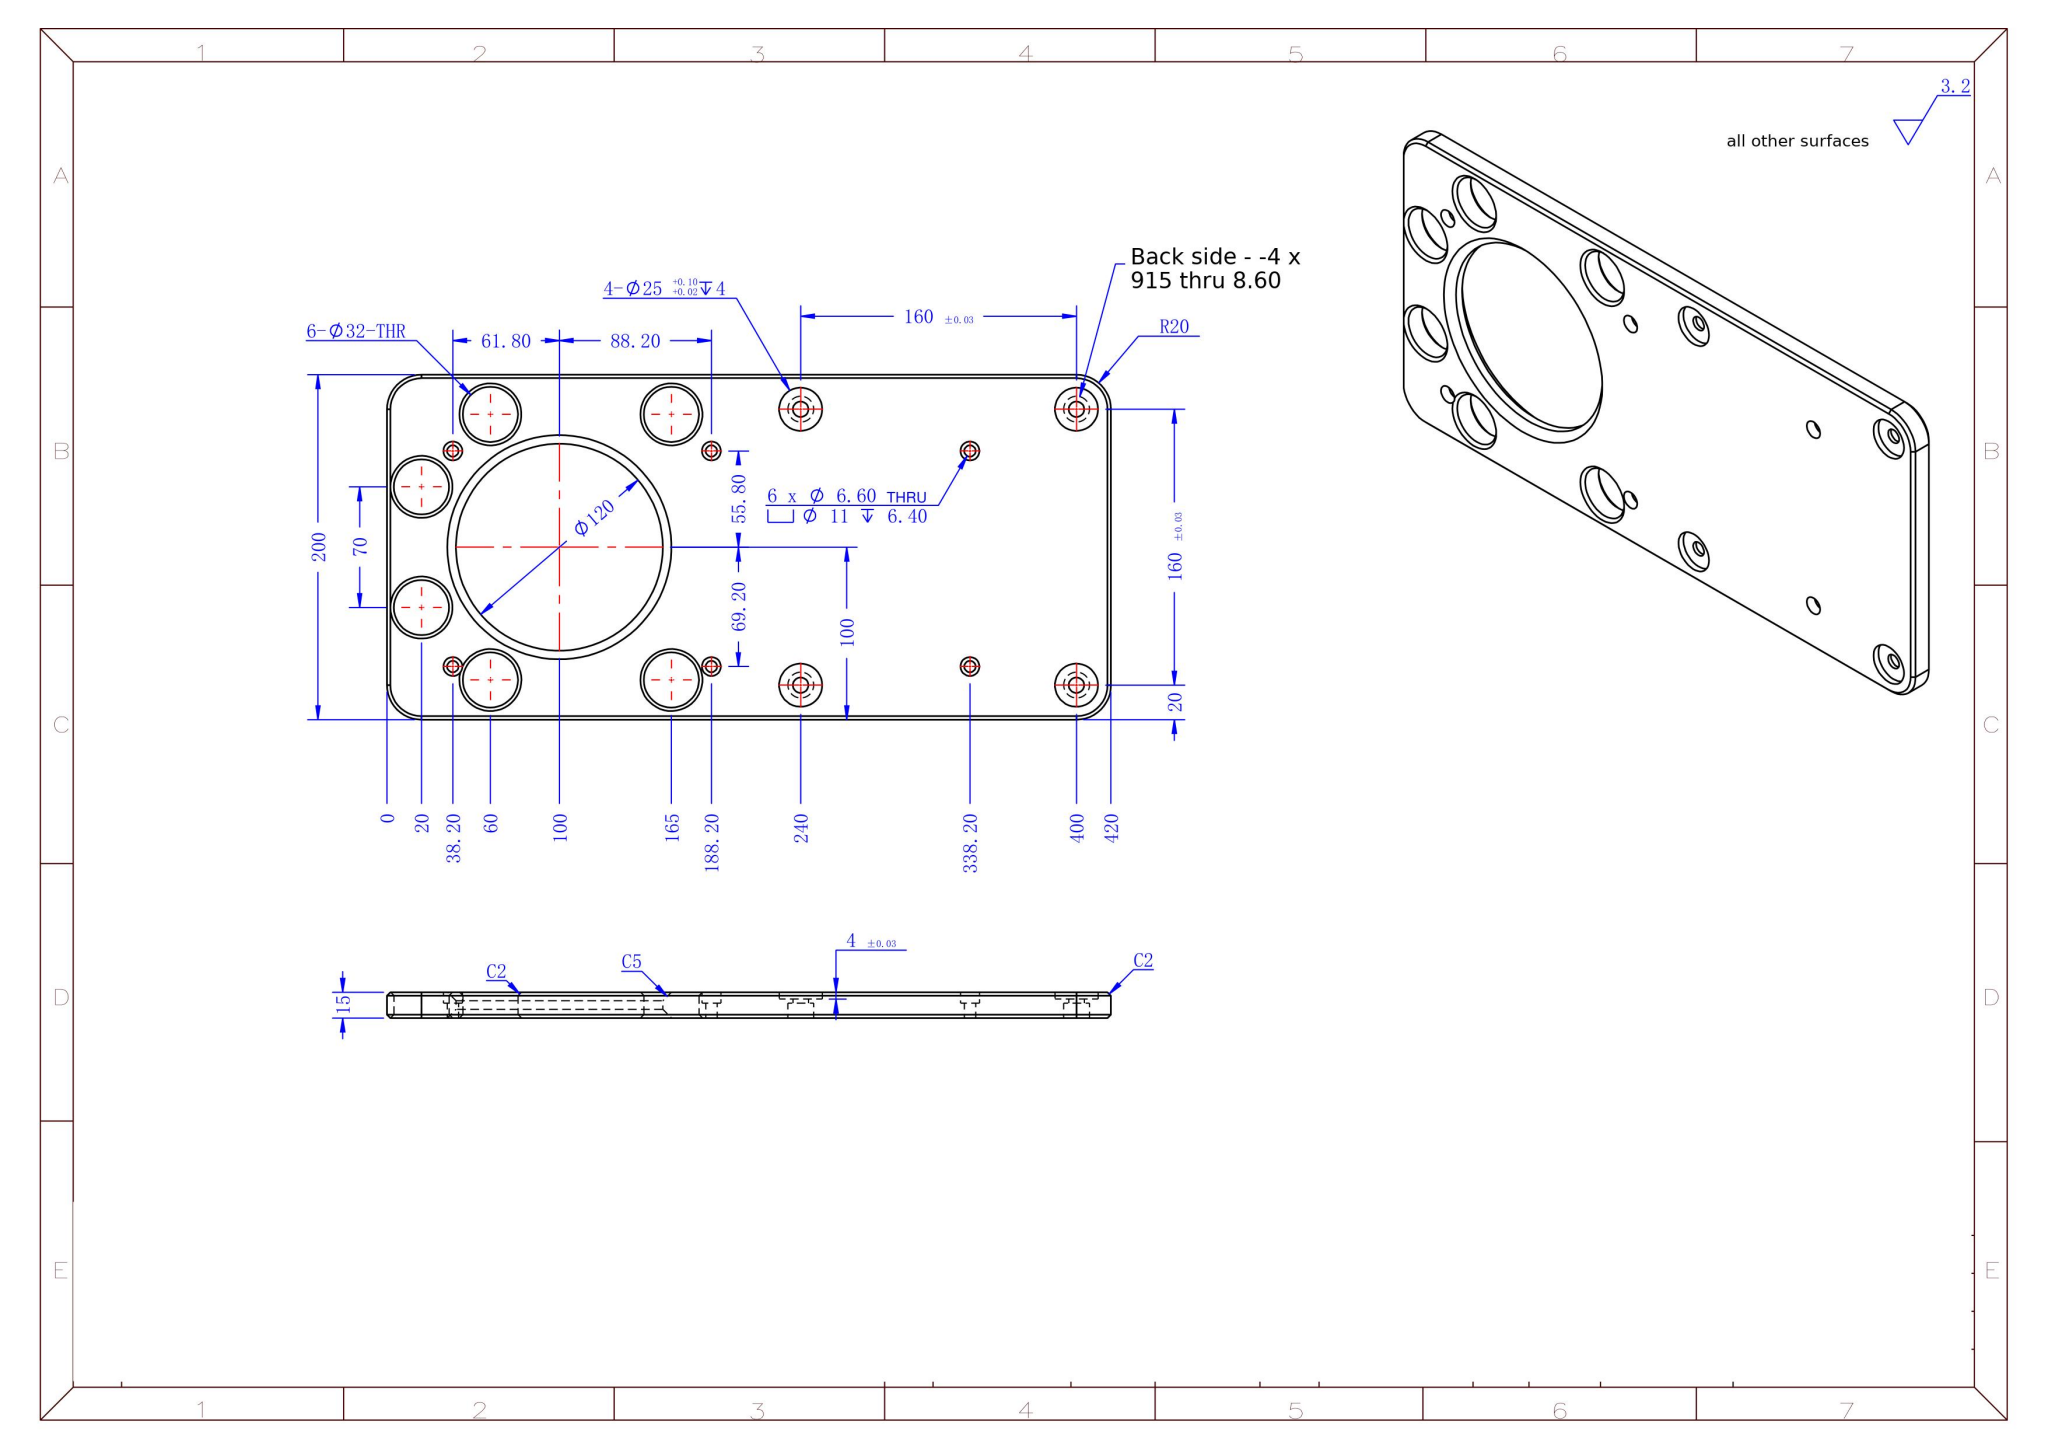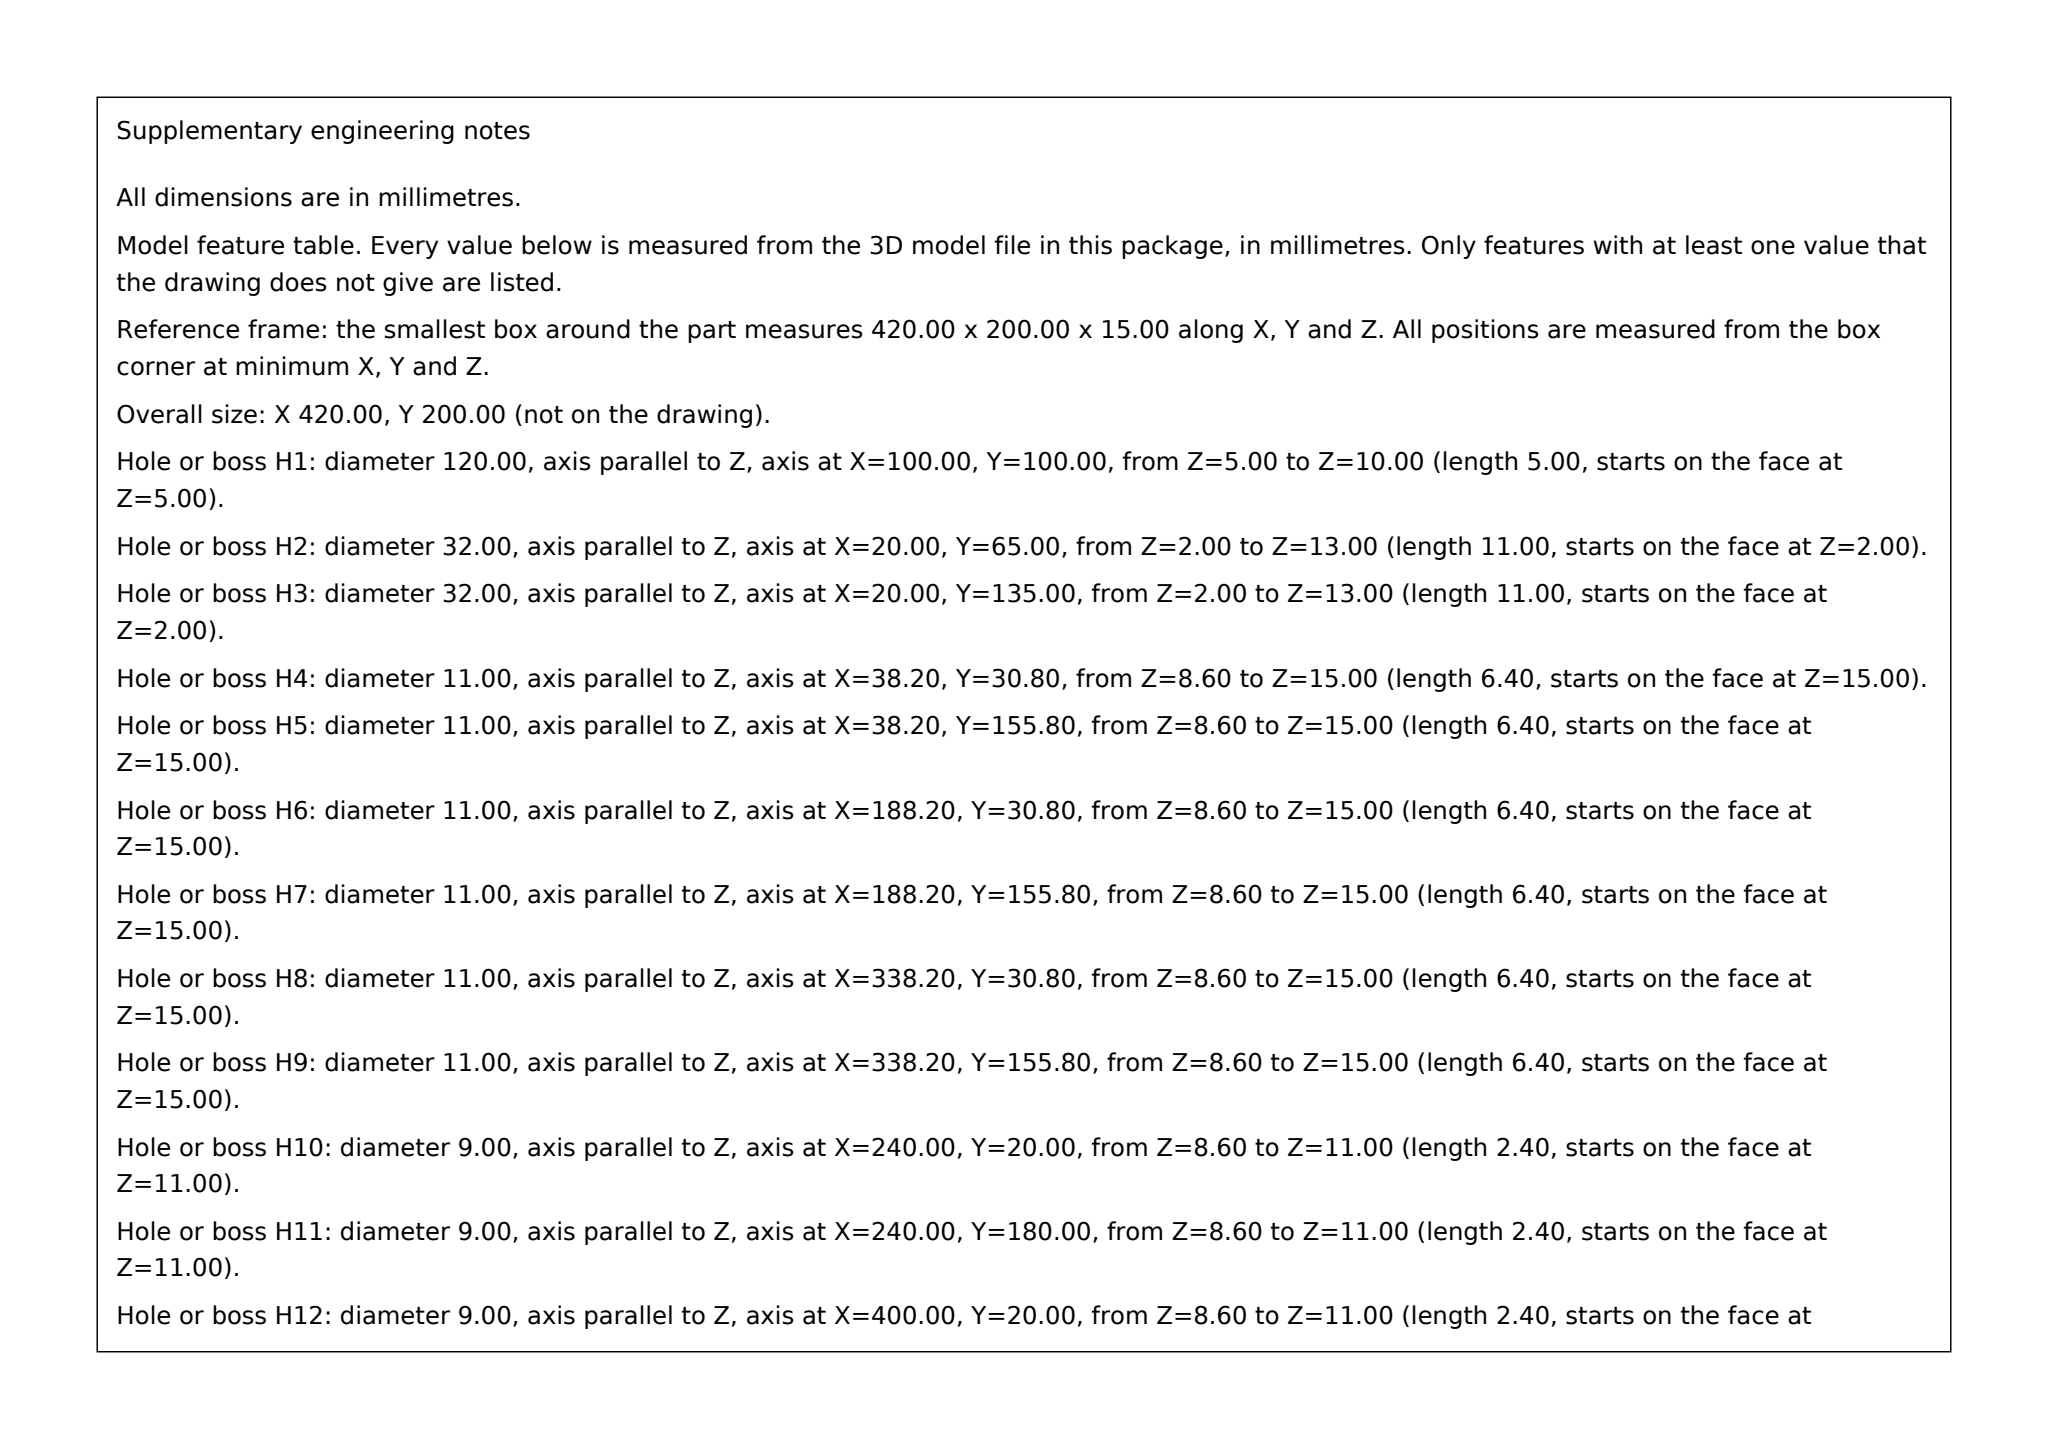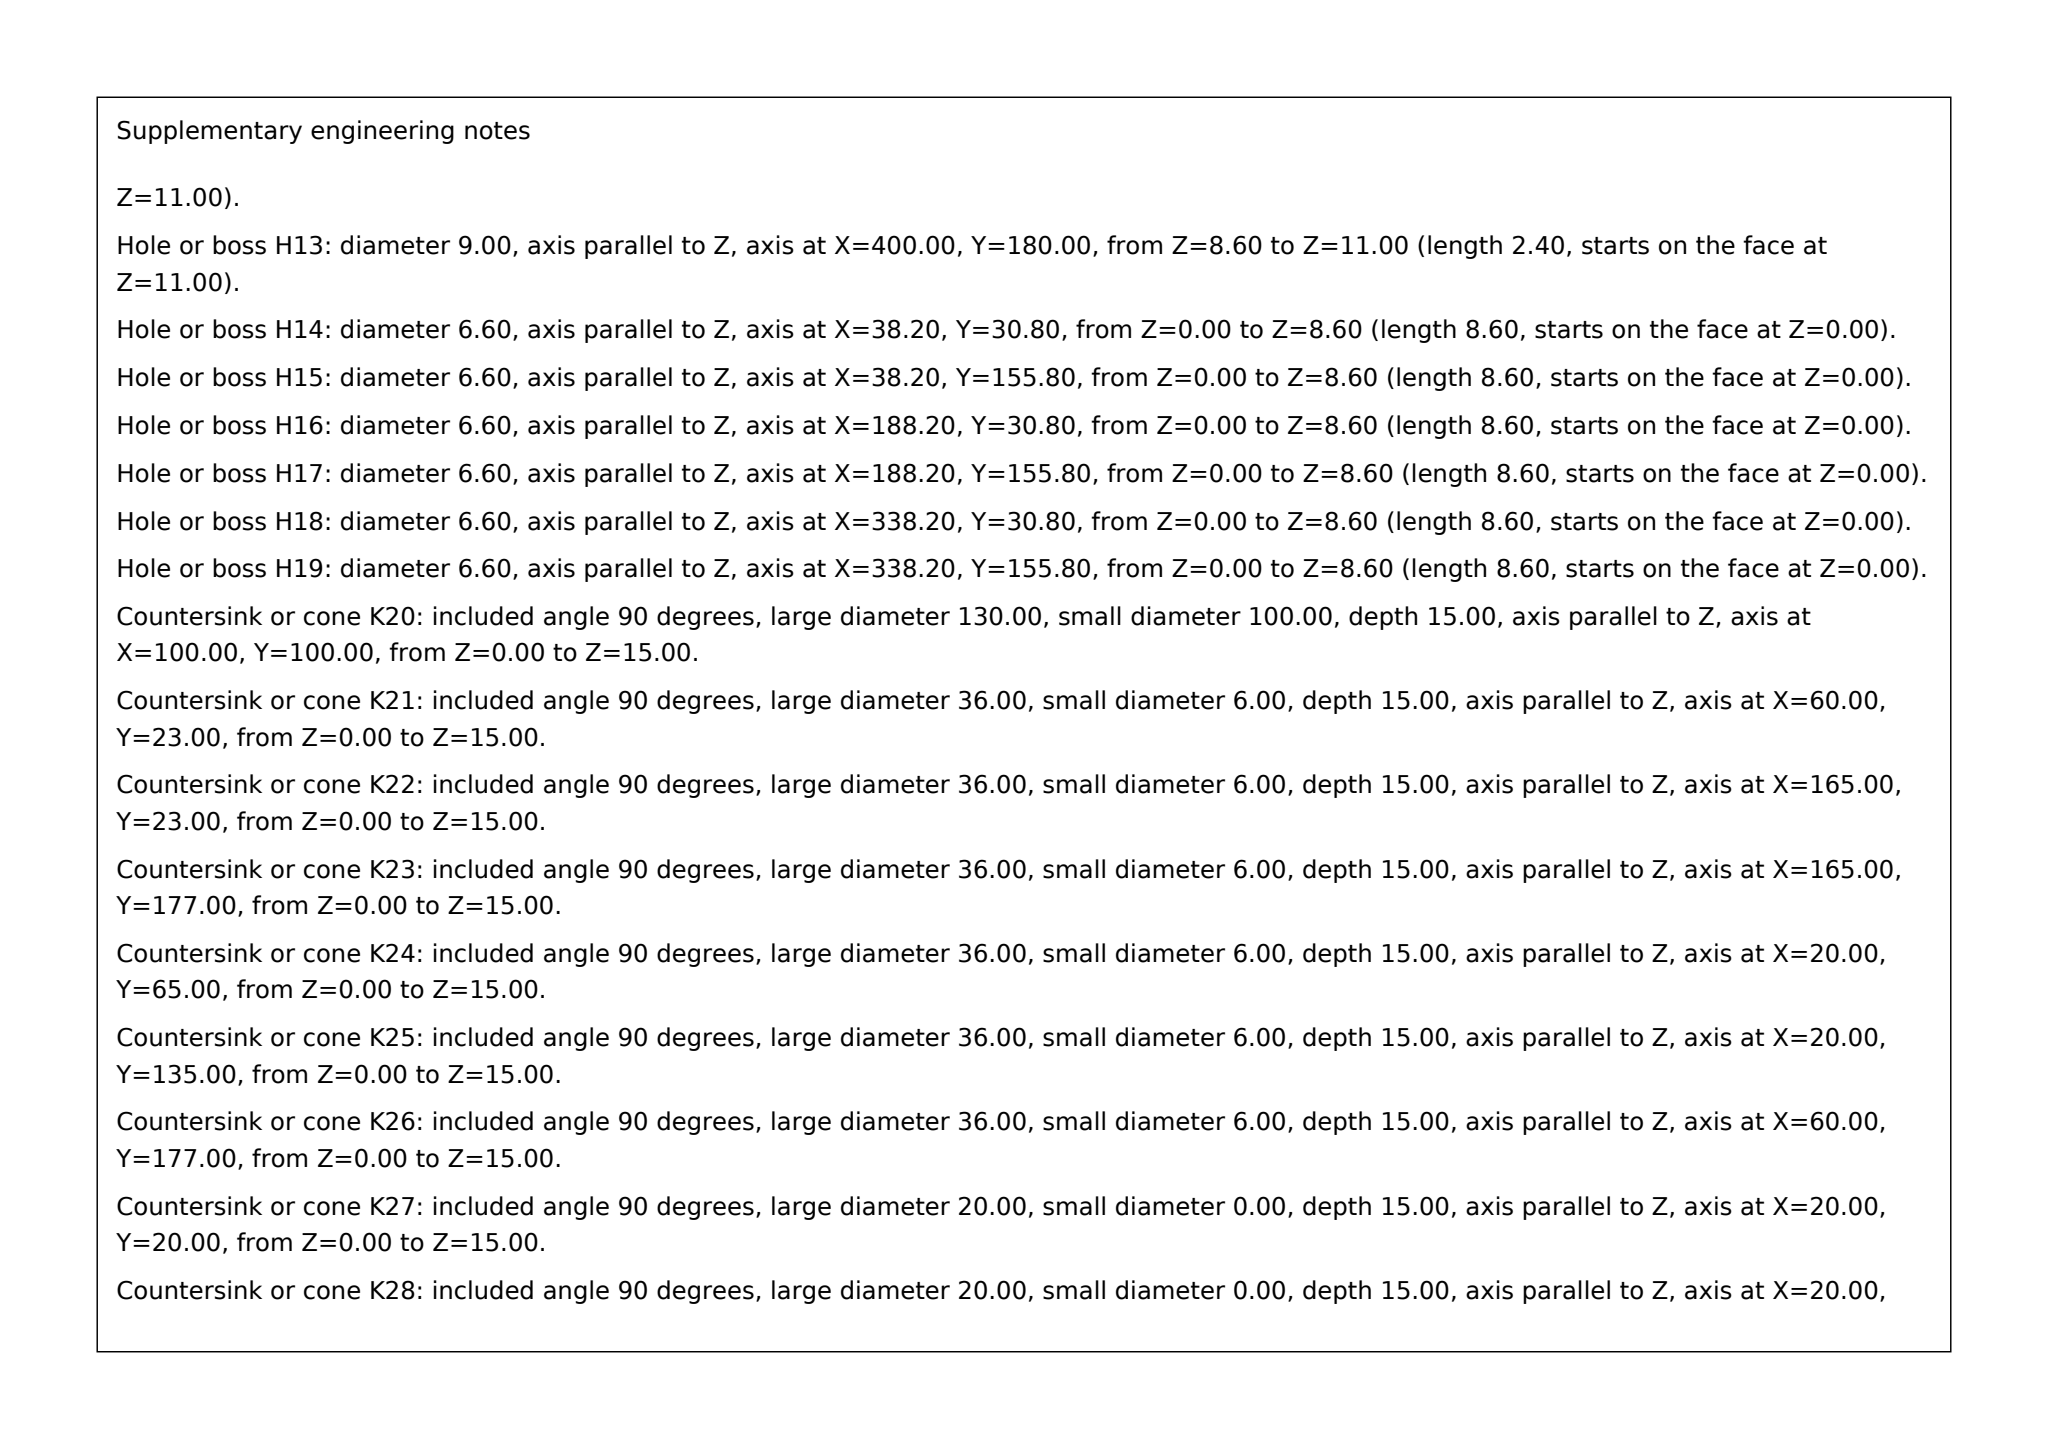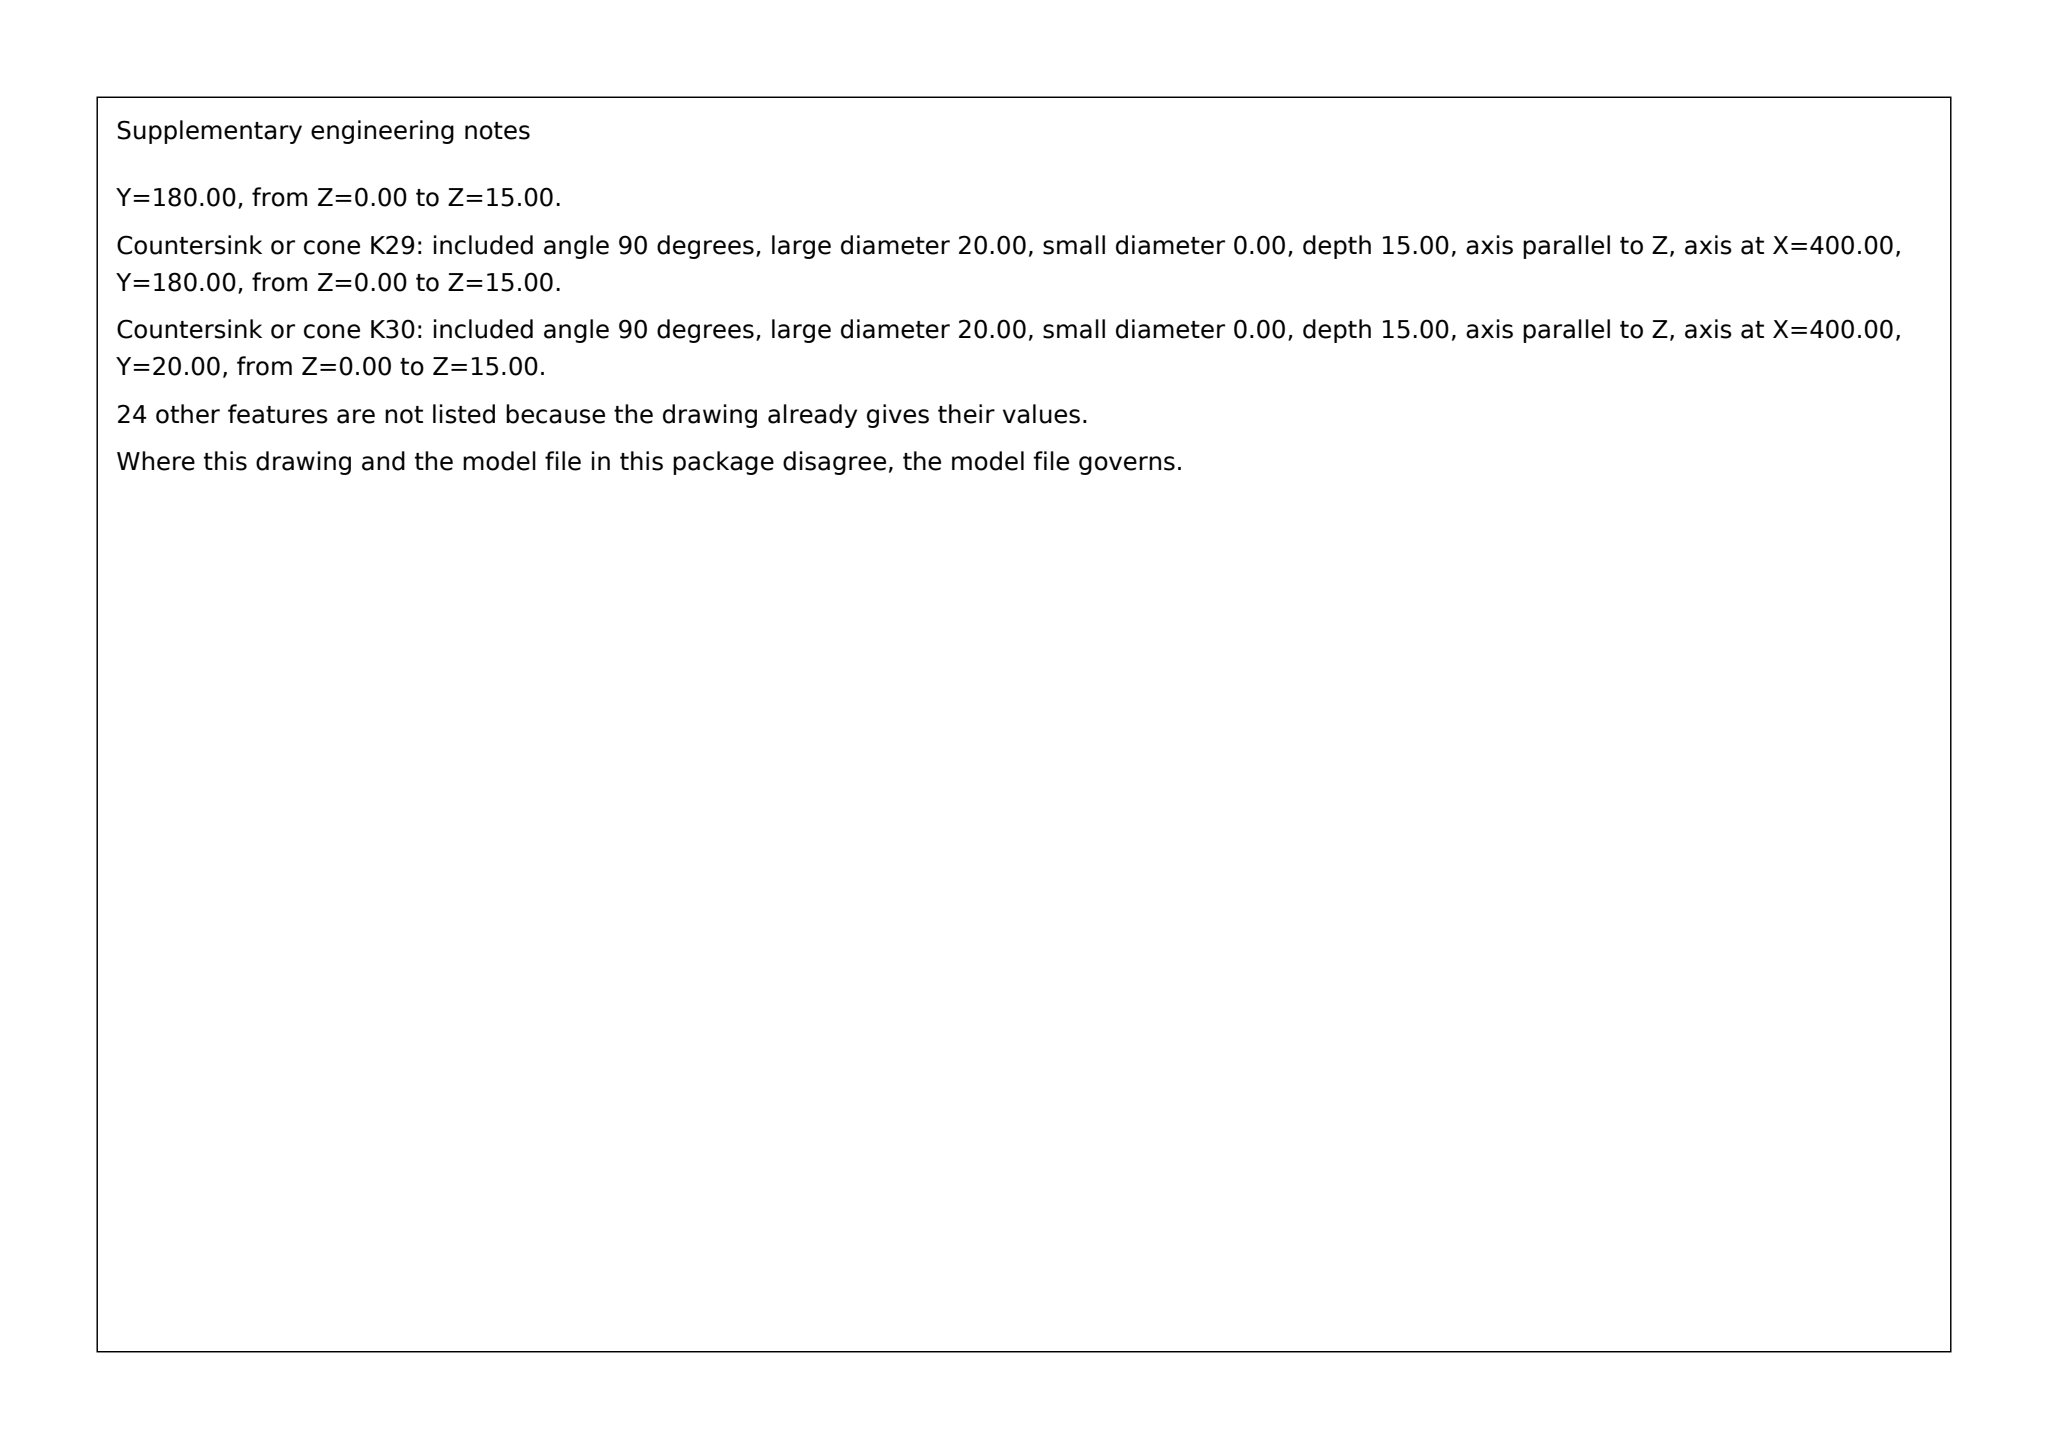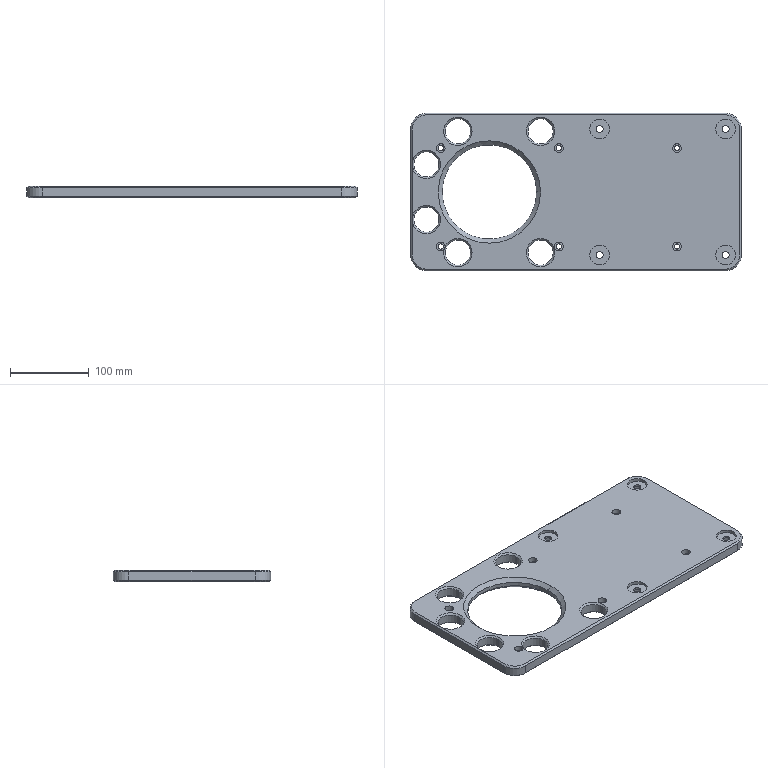Part | SolidWorks | mm | 1 solid | 130 faces | box 420 x 200 x 15 mm | volume 975857 mm3 | cylinder 66 | cone 36 | plane 28 | commonest cylinder face diameters 32 x12 11 x12 6.6 x12 15 x8 9 x8 25 x8 40 x4 120 x2